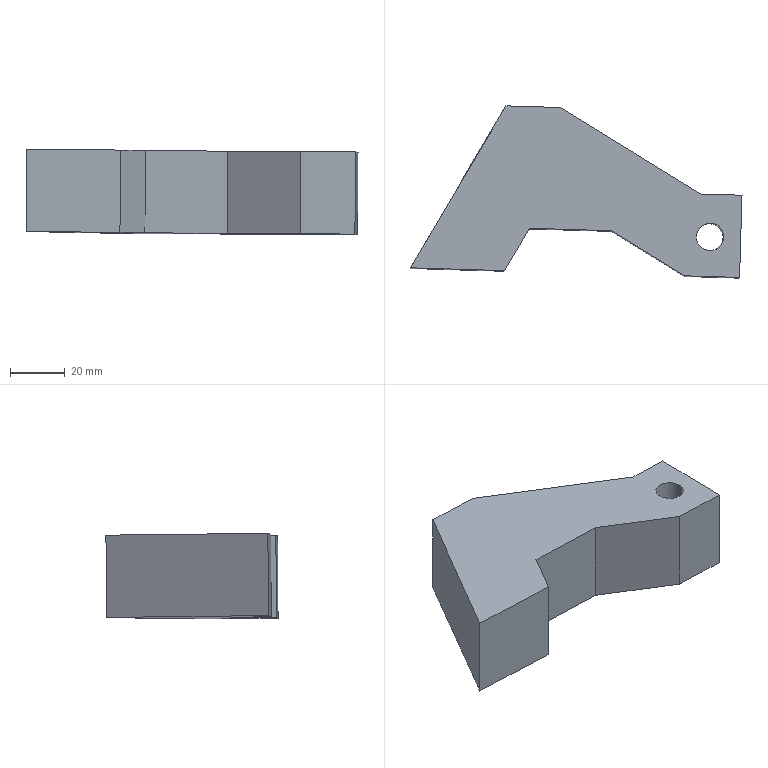Component | NX | M1002_AGO13_P09_757058_P01 | 1 solid | 13 faces | box 121.07 x 62.76 x 31.13 mm | volume 124638 mm3 | plane 12 | cylinder 1 | commonest cylinder face diameters 10 x1
STEP:
#1=CARTESIAN_POINT('',(0.,0.,0.));
#2=DIRECTION('',(0.,0.,1.));
#3=DIRECTION('',(1.,0.,0.));
#4=AXIS2_PLACEMENT_3D('',#1,#2,#3);
#5=CARTESIAN_POINT('',(-375.468,-402.725,117.7));
#6=VERTEX_POINT('',#5);
#7=CARTESIAN_POINT('',(-374.576,-372.739,117.492));
#8=VERTEX_POINT('',#7);
#9=CARTESIAN_POINT('',(-375.468,-402.725,117.7));
#10=DIRECTION('',(0.02973,0.9995,-0.006913));
#11=VECTOR('',#10,1.);
#12=LINE('',#9,#11);
#13=CARTESIAN_POINT('',(-375.23,-402.525,147.698));
#14=DIRECTION('',(-0.9995,0.02978,0.007726));
#15=DIRECTION('',(0.007929,0.00668,0.9999));
#16=AXIS2_PLACEMENT_3D('',#13,#14,#15);
#17=PLANE('',#16);
#18=CARTESIAN_POINT('',(-30.,-0.));
#19=DIRECTION('',(0.,1.));
#20=VECTOR('',#19,1.);
#21=LINE('',#18,#20);
#22=(GEOMETRIC_REPRESENTATION_CONTEXT(2)PARAMETRIC_REPRESENTATION_CONTEXT()REPRESENTATION_CONTEXT('',''));
#23=DEFINITIONAL_REPRESENTATION('',(#21),#22);
#24=PCURVE('',#17,#23);
#25=CARTESIAN_POINT('',(-386.232,-387.898,117.686));
#26=DIRECTION('',(0.007929,0.00668,0.9999));
#27=DIRECTION('',(0.9995,-0.02978,-0.007726));
#28=AXIS2_PLACEMENT_3D('',#25,#26,#27);
#29=PLANE('',#28);
#30=CARTESIAN_POINT('',(11.2,-14.5));
#31=DIRECTION('',(-0.,1.));
#32=VECTOR('',#31,1.);
#33=LINE('',#30,#32);
#34=(GEOMETRIC_REPRESENTATION_CONTEXT(2)PARAMETRIC_REPRESENTATION_CONTEXT()REPRESENTATION_CONTEXT('',''));
#35=DEFINITIONAL_REPRESENTATION('',(#33),#34);
#36=PCURVE('',#29,#35);
#37=SURFACE_CURVE('',#12,(#24,#36),.PCURVE_S1.);
#38=EDGE_CURVE('',#6,#8,#37,.T.);
#39=ORIENTED_EDGE('',*,*,#38,.T.);
#40=CARTESIAN_POINT('',(-374.338,-372.539,147.491));
#41=VERTEX_POINT('',#40);
#42=CARTESIAN_POINT('',(-374.338,-372.539,147.491));
#43=DIRECTION('',(-0.007929,-0.00668,-0.9999));
#44=VECTOR('',#43,1.);
#45=LINE('',#42,#44);
#46=CARTESIAN_POINT('',(-0.,30.));
#47=DIRECTION('',(-1.,0.));
#48=VECTOR('',#47,1.);
#49=LINE('',#46,#48);
#50=(GEOMETRIC_REPRESENTATION_CONTEXT(2)PARAMETRIC_REPRESENTATION_CONTEXT()REPRESENTATION_CONTEXT('',''));
#51=DEFINITIONAL_REPRESENTATION('',(#49),#50);
#52=PCURVE('',#17,#51);
#53=CARTESIAN_POINT('',(-374.338,-372.539,147.491));
#54=DIRECTION('',(-0.02973,-0.9995,0.006913));
#55=DIRECTION('',(0.9995,-0.02978,-0.007726));
#56=AXIS2_PLACEMENT_3D('',#53,#54,#55);
#57=PLANE('',#56);
#58=CARTESIAN_POINT('',(0.,0.));
#59=DIRECTION('',(-0.,-1.));
#60=VECTOR('',#59,1.);
#61=LINE('',#58,#60);
#62=(GEOMETRIC_REPRESENTATION_CONTEXT(2)PARAMETRIC_REPRESENTATION_CONTEXT()REPRESENTATION_CONTEXT('',''));
#63=DEFINITIONAL_REPRESENTATION('',(#61),#62);
#64=PCURVE('',#57,#63);
#65=SURFACE_CURVE('',#45,(#52,#64),.PCURVE_S1.);
#66=EDGE_CURVE('',#41,#8,#65,.T.);
#67=ORIENTED_EDGE('',*,*,#66,.F.);
#68=CARTESIAN_POINT('',(-375.23,-402.525,147.698));
#69=VERTEX_POINT('',#68);
#70=CARTESIAN_POINT('',(-375.23,-402.525,147.698));
#71=DIRECTION('',(0.02973,0.9995,-0.006913));
#72=VECTOR('',#71,1.);
#73=LINE('',#70,#72);
#74=CARTESIAN_POINT('',(0.,0.));
#75=DIRECTION('',(0.,1.));
#76=VECTOR('',#75,1.);
#77=LINE('',#74,#76);
#78=(GEOMETRIC_REPRESENTATION_CONTEXT(2)PARAMETRIC_REPRESENTATION_CONTEXT()REPRESENTATION_CONTEXT('',''));
#79=DEFINITIONAL_REPRESENTATION('',(#77),#78);
#80=PCURVE('',#17,#79);
#81=CARTESIAN_POINT('',(-385.994,-387.698,147.684));
#82=DIRECTION('',(0.007929,0.00668,0.9999));
#83=DIRECTION('',(0.9995,-0.02978,-0.007726));
#84=AXIS2_PLACEMENT_3D('',#81,#82,#83);
#85=PLANE('',#84);
#86=CARTESIAN_POINT('',(11.2,-14.5));
#87=DIRECTION('',(-0.,1.));
#88=VECTOR('',#87,1.);
#89=LINE('',#86,#88);
#90=(GEOMETRIC_REPRESENTATION_CONTEXT(2)PARAMETRIC_REPRESENTATION_CONTEXT()REPRESENTATION_CONTEXT('',''));
#91=DEFINITIONAL_REPRESENTATION('',(#89),#90);
#92=PCURVE('',#85,#91);
#93=SURFACE_CURVE('',#73,(#80,#92),.PCURVE_S1.);
#94=EDGE_CURVE('',#69,#41,#93,.T.);
#95=ORIENTED_EDGE('',*,*,#94,.F.);
#96=CARTESIAN_POINT('',(-375.23,-402.525,147.698));
#97=DIRECTION('',(-0.007929,-0.00668,-0.9999));
#98=VECTOR('',#97,1.);
#99=LINE('',#96,#98);
#100=CARTESIAN_POINT('',(0.,0.));
#101=DIRECTION('',(-1.,0.));
#102=VECTOR('',#101,1.);
#103=LINE('',#100,#102);
#104=(GEOMETRIC_REPRESENTATION_CONTEXT(2)PARAMETRIC_REPRESENTATION_CONTEXT()REPRESENTATION_CONTEXT('',''));
#105=DEFINITIONAL_REPRESENTATION('',(#103),#104);
#106=PCURVE('',#17,#105);
#107=CARTESIAN_POINT('',(-395.221,-401.929,147.853));
#108=DIRECTION('',(0.02973,0.9995,-0.006913));
#109=DIRECTION('',(-0.9995,0.02978,0.007726));
#110=AXIS2_PLACEMENT_3D('',#107,#108,#109);
#111=PLANE('',#110);
#112=CARTESIAN_POINT('',(-20.,-0.));
#113=DIRECTION('',(0.,-1.));
#114=VECTOR('',#113,1.);
#115=LINE('',#112,#114);
#116=(GEOMETRIC_REPRESENTATION_CONTEXT(2)PARAMETRIC_REPRESENTATION_CONTEXT()REPRESENTATION_CONTEXT('',''));
#117=DEFINITIONAL_REPRESENTATION('',(#115),#116);
#118=PCURVE('',#111,#117);
#119=SURFACE_CURVE('',#99,(#106,#118),.PCURVE_S1.);
#120=EDGE_CURVE('',#69,#6,#119,.T.);
#121=ORIENTED_EDGE('',*,*,#120,.T.);
#122=EDGE_LOOP('',(#39,#67,#95,#121));
#123=FACE_BOUND('',#122,.T.);
#124=ADVANCED_FACE('',(#123),#17,.F.);
#125=CARTESIAN_POINT('',(-389.569,-372.292,117.608));
#126=VERTEX_POINT('',#125);
#127=CARTESIAN_POINT('',(-374.576,-372.739,117.492));
#128=DIRECTION('',(-0.9995,0.02978,0.007726));
#129=VECTOR('',#128,1.);
#130=LINE('',#127,#129);
#131=CARTESIAN_POINT('',(-0.,-30.));
#132=DIRECTION('',(-1.,0.));
#133=VECTOR('',#132,1.);
#134=LINE('',#131,#133);
#135=(GEOMETRIC_REPRESENTATION_CONTEXT(2)PARAMETRIC_REPRESENTATION_CONTEXT()REPRESENTATION_CONTEXT('',''));
#136=DEFINITIONAL_REPRESENTATION('',(#134),#135);
#137=PCURVE('',#57,#136);
#138=CARTESIAN_POINT('',(11.2,15.5));
#139=DIRECTION('',(-1.,-0.));
#140=VECTOR('',#139,1.);
#141=LINE('',#138,#140);
#142=(GEOMETRIC_REPRESENTATION_CONTEXT(2)PARAMETRIC_REPRESENTATION_CONTEXT()REPRESENTATION_CONTEXT('',''));
#143=DEFINITIONAL_REPRESENTATION('',(#141),#142);
#144=PCURVE('',#29,#143);
#145=SURFACE_CURVE('',#130,(#137,#144),.PCURVE_S1.);
#146=EDGE_CURVE('',#8,#126,#145,.T.);
#147=ORIENTED_EDGE('',*,*,#146,.T.);
#148=CARTESIAN_POINT('',(-389.331,-372.092,147.607));
#149=VERTEX_POINT('',#148);
#150=CARTESIAN_POINT('',(-389.331,-372.092,147.607));
#151=DIRECTION('',(-0.007929,-0.00668,-0.9999));
#152=VECTOR('',#151,1.);
#153=LINE('',#150,#152);
#154=CARTESIAN_POINT('',(-15.,0.));
#155=DIRECTION('',(-0.,-1.));
#156=VECTOR('',#155,1.);
#157=LINE('',#154,#156);
#158=(GEOMETRIC_REPRESENTATION_CONTEXT(2)PARAMETRIC_REPRESENTATION_CONTEXT()REPRESENTATION_CONTEXT('',''));
#159=DEFINITIONAL_REPRESENTATION('',(#157),#158);
#160=PCURVE('',#57,#159);
#161=CARTESIAN_POINT('',(-389.331,-372.092,147.607));
#162=DIRECTION('',(-0.5252,-0.8509,0.009849));
#163=DIRECTION('',(0.8509,-0.5253,-0.003238));
#164=AXIS2_PLACEMENT_3D('',#161,#162,#163);
#165=PLANE('',#164);
#166=CARTESIAN_POINT('',(0.,0.));
#167=DIRECTION('',(0.,-1.));
#168=VECTOR('',#167,1.);
#169=LINE('',#166,#168);
#170=(GEOMETRIC_REPRESENTATION_CONTEXT(2)PARAMETRIC_REPRESENTATION_CONTEXT()REPRESENTATION_CONTEXT('',''));
#171=DEFINITIONAL_REPRESENTATION('',(#169),#170);
#172=PCURVE('',#165,#171);
#173=SURFACE_CURVE('',#153,(#160,#172),.PCURVE_S1.);
#174=EDGE_CURVE('',#149,#126,#173,.T.);
#175=ORIENTED_EDGE('',*,*,#174,.F.);
#176=CARTESIAN_POINT('',(-374.338,-372.539,147.491));
#177=DIRECTION('',(-0.9995,0.02978,0.007726));
#178=VECTOR('',#177,1.);
#179=LINE('',#176,#178);
#180=CARTESIAN_POINT('',(0.,0.));
#181=DIRECTION('',(-1.,0.));
#182=VECTOR('',#181,1.);
#183=LINE('',#180,#182);
#184=(GEOMETRIC_REPRESENTATION_CONTEXT(2)PARAMETRIC_REPRESENTATION_CONTEXT()REPRESENTATION_CONTEXT('',''));
#185=DEFINITIONAL_REPRESENTATION('',(#183),#184);
#186=PCURVE('',#57,#185);
#187=CARTESIAN_POINT('',(11.2,15.5));
#188=DIRECTION('',(-1.,-0.));
#189=VECTOR('',#188,1.);
#190=LINE('',#187,#189);
#191=(GEOMETRIC_REPRESENTATION_CONTEXT(2)PARAMETRIC_REPRESENTATION_CONTEXT()REPRESENTATION_CONTEXT('',''));
#192=DEFINITIONAL_REPRESENTATION('',(#190),#191);
#193=PCURVE('',#85,#192);
#194=SURFACE_CURVE('',#179,(#186,#193),.PCURVE_S1.);
#195=EDGE_CURVE('',#41,#149,#194,.T.);
#196=ORIENTED_EDGE('',*,*,#195,.F.);
#197=ORIENTED_EDGE('',*,*,#66,.T.);
#198=EDGE_LOOP('',(#147,#175,#196,#197));
#199=FACE_BOUND('',#198,.T.);
#200=ADVANCED_FACE('',(#199),#57,.F.);
#201=CARTESIAN_POINT('',(-440.653,-340.758,117.803));
#202=VERTEX_POINT('',#201);
#203=CARTESIAN_POINT('',(-389.569,-372.292,117.608));
#204=DIRECTION('',(-0.8509,0.5253,0.003238));
#205=VECTOR('',#204,1.);
#206=LINE('',#203,#205);
#207=CARTESIAN_POINT('',(0.,-30.));
#208=DIRECTION('',(-1.,-0.));
#209=VECTOR('',#208,1.);
#210=LINE('',#207,#209);
#211=(GEOMETRIC_REPRESENTATION_CONTEXT(2)PARAMETRIC_REPRESENTATION_CONTEXT()REPRESENTATION_CONTEXT('',''));
#212=DEFINITIONAL_REPRESENTATION('',(#210),#211);
#213=PCURVE('',#165,#212);
#214=CARTESIAN_POINT('',(-3.8,15.5));
#215=DIRECTION('',(-0.8662,0.4997));
#216=VECTOR('',#215,1.);
#217=LINE('',#214,#216);
#218=(GEOMETRIC_REPRESENTATION_CONTEXT(2)PARAMETRIC_REPRESENTATION_CONTEXT()REPRESENTATION_CONTEXT('',''));
#219=DEFINITIONAL_REPRESENTATION('',(#217),#218);
#220=PCURVE('',#29,#219);
#221=SURFACE_CURVE('',#206,(#213,#220),.PCURVE_S1.);
#222=EDGE_CURVE('',#126,#202,#221,.T.);
#223=ORIENTED_EDGE('',*,*,#222,.T.);
#224=CARTESIAN_POINT('',(-440.415,-340.557,147.801));
#225=VERTEX_POINT('',#224);
#226=CARTESIAN_POINT('',(-440.415,-340.557,147.801));
#227=DIRECTION('',(-0.007929,-0.00668,-0.9999));
#228=VECTOR('',#227,1.);
#229=LINE('',#226,#228);
#230=CARTESIAN_POINT('',(-60.033,-0.));
#231=DIRECTION('',(0.,-1.));
#232=VECTOR('',#231,1.);
#233=LINE('',#230,#232);
#234=(GEOMETRIC_REPRESENTATION_CONTEXT(2)PARAMETRIC_REPRESENTATION_CONTEXT()REPRESENTATION_CONTEXT('',''));
#235=DEFINITIONAL_REPRESENTATION('',(#233),#234);
#236=PCURVE('',#165,#235);
#237=CARTESIAN_POINT('',(-440.415,-340.557,147.801));
#238=DIRECTION('',(-0.02973,-0.9995,0.006913));
#239=DIRECTION('',(0.9995,-0.02978,-0.007726));
#240=AXIS2_PLACEMENT_3D('',#237,#238,#239);
#241=PLANE('',#240);
#242=CARTESIAN_POINT('',(0.,0.));
#243=DIRECTION('',(-0.,-1.));
#244=VECTOR('',#243,1.);
#245=LINE('',#242,#244);
#246=(GEOMETRIC_REPRESENTATION_CONTEXT(2)PARAMETRIC_REPRESENTATION_CONTEXT()REPRESENTATION_CONTEXT('',''));
#247=DEFINITIONAL_REPRESENTATION('',(#245),#246);
#248=PCURVE('',#241,#247);
#249=SURFACE_CURVE('',#229,(#236,#248),.PCURVE_S1.);
#250=EDGE_CURVE('',#225,#202,#249,.T.);
#251=ORIENTED_EDGE('',*,*,#250,.F.);
#252=CARTESIAN_POINT('',(-389.331,-372.092,147.607));
#253=DIRECTION('',(-0.8509,0.5253,0.003238));
#254=VECTOR('',#253,1.);
#255=LINE('',#252,#254);
#256=CARTESIAN_POINT('',(0.,0.));
#257=DIRECTION('',(-1.,-0.));
#258=VECTOR('',#257,1.);
#259=LINE('',#256,#258);
#260=(GEOMETRIC_REPRESENTATION_CONTEXT(2)PARAMETRIC_REPRESENTATION_CONTEXT()REPRESENTATION_CONTEXT('',''));
#261=DEFINITIONAL_REPRESENTATION('',(#259),#260);
#262=PCURVE('',#165,#261);
#263=CARTESIAN_POINT('',(-3.8,15.5));
#264=DIRECTION('',(-0.8662,0.4997));
#265=VECTOR('',#264,1.);
#266=LINE('',#263,#265);
#267=(GEOMETRIC_REPRESENTATION_CONTEXT(2)PARAMETRIC_REPRESENTATION_CONTEXT()REPRESENTATION_CONTEXT('',''));
#268=DEFINITIONAL_REPRESENTATION('',(#266),#267);
#269=PCURVE('',#85,#268);
#270=SURFACE_CURVE('',#255,(#262,#269),.PCURVE_S1.);
#271=EDGE_CURVE('',#149,#225,#270,.T.);
#272=ORIENTED_EDGE('',*,*,#271,.F.);
#273=ORIENTED_EDGE('',*,*,#174,.T.);
#274=EDGE_LOOP('',(#223,#251,#272,#273));
#275=FACE_BOUND('',#274,.T.);
#276=ADVANCED_FACE('',(#275),#165,.F.);
#277=CARTESIAN_POINT('',(-460.643,-340.162,117.957));
#278=VERTEX_POINT('',#277);
#279=CARTESIAN_POINT('',(-440.653,-340.758,117.803));
#280=DIRECTION('',(-0.9995,0.02978,0.007726));
#281=VECTOR('',#280,1.);
#282=LINE('',#279,#281);
#283=CARTESIAN_POINT('',(-0.,-30.));
#284=DIRECTION('',(-1.,0.));
#285=VECTOR('',#284,1.);
#286=LINE('',#283,#285);
#287=(GEOMETRIC_REPRESENTATION_CONTEXT(2)PARAMETRIC_REPRESENTATION_CONTEXT()REPRESENTATION_CONTEXT('',''));
#288=DEFINITIONAL_REPRESENTATION('',(#286),#287);
#289=PCURVE('',#241,#288);
#290=CARTESIAN_POINT('',(-55.8,45.5));
#291=DIRECTION('',(-1.,-0.));
#292=VECTOR('',#291,1.);
#293=LINE('',#290,#292);
#294=(GEOMETRIC_REPRESENTATION_CONTEXT(2)PARAMETRIC_REPRESENTATION_CONTEXT()REPRESENTATION_CONTEXT('',''));
#295=DEFINITIONAL_REPRESENTATION('',(#293),#294);
#296=PCURVE('',#29,#295);
#297=SURFACE_CURVE('',#282,(#289,#296),.PCURVE_S1.);
#298=EDGE_CURVE('',#202,#278,#297,.T.);
#299=ORIENTED_EDGE('',*,*,#298,.T.);
#300=CARTESIAN_POINT('',(-460.405,-339.962,147.956));
#301=VERTEX_POINT('',#300);
#302=CARTESIAN_POINT('',(-460.405,-339.962,147.956));
#303=DIRECTION('',(-0.007929,-0.00668,-0.9999));
#304=VECTOR('',#303,1.);
#305=LINE('',#302,#304);
#306=CARTESIAN_POINT('',(-20.,-0.));
#307=DIRECTION('',(-0.,-1.));
#308=VECTOR('',#307,1.);
#309=LINE('',#306,#308);
#310=(GEOMETRIC_REPRESENTATION_CONTEXT(2)PARAMETRIC_REPRESENTATION_CONTEXT()REPRESENTATION_CONTEXT('',''));
#311=DEFINITIONAL_REPRESENTATION('',(#309),#310);
#312=PCURVE('',#241,#311);
#313=CARTESIAN_POINT('',(-460.405,-339.962,147.956));
#314=DIRECTION('',(0.8617,-0.5074,-0.003443));
#315=DIRECTION('',(0.5073,0.8617,-0.00978));
#316=AXIS2_PLACEMENT_3D('',#313,#314,#315);
#317=PLANE('',#316);
#318=CARTESIAN_POINT('',(0.,0.));
#319=DIRECTION('',(0.,-1.));
#320=VECTOR('',#319,1.);
#321=LINE('',#318,#320);
#322=(GEOMETRIC_REPRESENTATION_CONTEXT(2)PARAMETRIC_REPRESENTATION_CONTEXT()REPRESENTATION_CONTEXT('',''));
#323=DEFINITIONAL_REPRESENTATION('',(#321),#322);
#324=PCURVE('',#317,#323);
#325=SURFACE_CURVE('',#305,(#312,#324),.PCURVE_S1.);
#326=EDGE_CURVE('',#301,#278,#325,.T.);
#327=ORIENTED_EDGE('',*,*,#326,.F.);
#328=CARTESIAN_POINT('',(-440.415,-340.557,147.801));
#329=DIRECTION('',(-0.9995,0.02978,0.007726));
#330=VECTOR('',#329,1.);
#331=LINE('',#328,#330);
#332=CARTESIAN_POINT('',(0.,0.));
#333=DIRECTION('',(-1.,0.));
#334=VECTOR('',#333,1.);
#335=LINE('',#332,#334);
#336=(GEOMETRIC_REPRESENTATION_CONTEXT(2)PARAMETRIC_REPRESENTATION_CONTEXT()REPRESENTATION_CONTEXT('',''));
#337=DEFINITIONAL_REPRESENTATION('',(#335),#336);
#338=PCURVE('',#241,#337);
#339=CARTESIAN_POINT('',(-55.8,45.5));
#340=DIRECTION('',(-1.,-0.));
#341=VECTOR('',#340,1.);
#342=LINE('',#339,#341);
#343=(GEOMETRIC_REPRESENTATION_CONTEXT(2)PARAMETRIC_REPRESENTATION_CONTEXT()REPRESENTATION_CONTEXT('',''));
#344=DEFINITIONAL_REPRESENTATION('',(#342),#343);
#345=PCURVE('',#85,#344);
#346=SURFACE_CURVE('',#331,(#338,#345),.PCURVE_S1.);
#347=EDGE_CURVE('',#225,#301,#346,.T.);
#348=ORIENTED_EDGE('',*,*,#347,.F.);
#349=ORIENTED_EDGE('',*,*,#250,.T.);
#350=EDGE_LOOP('',(#299,#327,#348,#349));
#351=FACE_BOUND('',#350,.T.);
#352=ADVANCED_FACE('',(#351),#241,.F.);
#353=CARTESIAN_POINT('',(-495.413,-399.217,118.627));
#354=VERTEX_POINT('',#353);
#355=CARTESIAN_POINT('',(-460.643,-340.162,117.957));
#356=DIRECTION('',(-0.5073,-0.8617,0.00978));
#357=VECTOR('',#356,1.);
#358=LINE('',#355,#357);
#359=CARTESIAN_POINT('',(0.,-30.));
#360=DIRECTION('',(-1.,-0.));
#361=VECTOR('',#360,1.);
#362=LINE('',#359,#361);
#363=(GEOMETRIC_REPRESENTATION_CONTEXT(2)PARAMETRIC_REPRESENTATION_CONTEXT()REPRESENTATION_CONTEXT('',''));
#364=DEFINITIONAL_REPRESENTATION('',(#362),#363);
#365=PCURVE('',#317,#364);
#366=CARTESIAN_POINT('',(-75.8,45.5));
#367=DIRECTION('',(-0.4815,-0.8764));
#368=VECTOR('',#367,1.);
#369=LINE('',#366,#368);
#370=(GEOMETRIC_REPRESENTATION_CONTEXT(2)PARAMETRIC_REPRESENTATION_CONTEXT()REPRESENTATION_CONTEXT('',''));
#371=DEFINITIONAL_REPRESENTATION('',(#369),#370);
#372=PCURVE('',#29,#371);
#373=SURFACE_CURVE('',#358,(#365,#372),.PCURVE_S1.);
#374=EDGE_CURVE('',#278,#354,#373,.T.);
#375=ORIENTED_EDGE('',*,*,#374,.T.);
#376=CARTESIAN_POINT('',(-495.175,-399.017,148.626));
#377=VERTEX_POINT('',#376);
#378=CARTESIAN_POINT('',(-495.175,-399.017,148.626));
#379=DIRECTION('',(-0.007929,-0.00668,-0.9999));
#380=VECTOR('',#379,1.);
#381=LINE('',#378,#380);
#382=CARTESIAN_POINT('',(-68.534,-0.));
#383=DIRECTION('',(0.,-1.));
#384=VECTOR('',#383,1.);
#385=LINE('',#382,#384);
#386=(GEOMETRIC_REPRESENTATION_CONTEXT(2)PARAMETRIC_REPRESENTATION_CONTEXT()REPRESENTATION_CONTEXT('',''));
#387=DEFINITIONAL_REPRESENTATION('',(#385),#386);
#388=PCURVE('',#317,#387);
#389=CARTESIAN_POINT('',(-495.175,-399.017,148.626));
#390=DIRECTION('',(0.02973,0.9995,-0.006913));
#391=DIRECTION('',(-0.9995,0.02978,0.007726));
#392=AXIS2_PLACEMENT_3D('',#389,#390,#391);
#393=PLANE('',#392);
#394=CARTESIAN_POINT('',(0.,0.));
#395=DIRECTION('',(0.,-1.));
#396=VECTOR('',#395,1.);
#397=LINE('',#394,#396);
#398=(GEOMETRIC_REPRESENTATION_CONTEXT(2)PARAMETRIC_REPRESENTATION_CONTEXT()REPRESENTATION_CONTEXT('',''));
#399=DEFINITIONAL_REPRESENTATION('',(#397),#398);
#400=PCURVE('',#393,#399);
#401=SURFACE_CURVE('',#381,(#388,#400),.PCURVE_S1.);
#402=EDGE_CURVE('',#377,#354,#401,.T.);
#403=ORIENTED_EDGE('',*,*,#402,.F.);
#404=CARTESIAN_POINT('',(-460.405,-339.962,147.956));
#405=DIRECTION('',(-0.5073,-0.8617,0.00978));
#406=VECTOR('',#405,1.);
#407=LINE('',#404,#406);
#408=CARTESIAN_POINT('',(0.,0.));
#409=DIRECTION('',(-1.,-0.));
#410=VECTOR('',#409,1.);
#411=LINE('',#408,#410);
#412=(GEOMETRIC_REPRESENTATION_CONTEXT(2)PARAMETRIC_REPRESENTATION_CONTEXT()REPRESENTATION_CONTEXT('',''));
#413=DEFINITIONAL_REPRESENTATION('',(#411),#412);
#414=PCURVE('',#317,#413);
#415=CARTESIAN_POINT('',(-75.8,45.5));
#416=DIRECTION('',(-0.4815,-0.8764));
#417=VECTOR('',#416,1.);
#418=LINE('',#415,#417);
#419=(GEOMETRIC_REPRESENTATION_CONTEXT(2)PARAMETRIC_REPRESENTATION_CONTEXT()REPRESENTATION_CONTEXT('',''));
#420=DEFINITIONAL_REPRESENTATION('',(#418),#419);
#421=PCURVE('',#85,#420);
#422=SURFACE_CURVE('',#407,(#414,#421),.PCURVE_S1.);
#423=EDGE_CURVE('',#301,#377,#422,.T.);
#424=ORIENTED_EDGE('',*,*,#423,.F.);
#425=ORIENTED_EDGE('',*,*,#326,.T.);
#426=EDGE_LOOP('',(#375,#403,#424,#425));
#427=FACE_BOUND('',#426,.T.);
#428=ADVANCED_FACE('',(#427),#317,.F.);
#429=CARTESIAN_POINT('',(-461.155,-400.238,118.363));
#430=VERTEX_POINT('',#429);
#431=CARTESIAN_POINT('',(-495.413,-399.217,118.627));
#432=DIRECTION('',(0.9995,-0.02978,-0.007726));
#433=VECTOR('',#432,1.);
#434=LINE('',#431,#433);
#435=CARTESIAN_POINT('',(0.,-30.));
#436=DIRECTION('',(-1.,-0.));
#437=VECTOR('',#436,1.);
#438=LINE('',#435,#437);
#439=(GEOMETRIC_REPRESENTATION_CONTEXT(2)PARAMETRIC_REPRESENTATION_CONTEXT()REPRESENTATION_CONTEXT('',''));
#440=DEFINITIONAL_REPRESENTATION('',(#438),#439);
#441=PCURVE('',#393,#440);
#442=CARTESIAN_POINT('',(-108.8,-14.565));
#443=DIRECTION('',(1.,0.));
#444=VECTOR('',#443,1.);
#445=LINE('',#442,#444);
#446=(GEOMETRIC_REPRESENTATION_CONTEXT(2)PARAMETRIC_REPRESENTATION_CONTEXT()REPRESENTATION_CONTEXT('',''));
#447=DEFINITIONAL_REPRESENTATION('',(#445),#446);
#448=PCURVE('',#29,#447);
#449=SURFACE_CURVE('',#434,(#441,#448),.PCURVE_S1.);
#450=EDGE_CURVE('',#354,#430,#449,.T.);
#451=ORIENTED_EDGE('',*,*,#450,.T.);
#452=CARTESIAN_POINT('',(-460.917,-400.037,148.361));
#453=VERTEX_POINT('',#452);
#454=CARTESIAN_POINT('',(-460.917,-400.037,148.361));
#455=DIRECTION('',(-0.007929,-0.00668,-0.9999));
#456=VECTOR('',#455,1.);
#457=LINE('',#454,#456);
#458=CARTESIAN_POINT('',(-34.274,0.));
#459=DIRECTION('',(0.,-1.));
#460=VECTOR('',#459,1.);
#461=LINE('',#458,#460);
#462=(GEOMETRIC_REPRESENTATION_CONTEXT(2)PARAMETRIC_REPRESENTATION_CONTEXT()REPRESENTATION_CONTEXT('',''));
#463=DEFINITIONAL_REPRESENTATION('',(#461),#462);
#464=PCURVE('',#393,#463);
#465=CARTESIAN_POINT('',(-460.917,-400.037,148.361));
#466=DIRECTION('',(-0.8617,0.5074,0.003443));
#467=DIRECTION('',(-0.5073,-0.8617,0.00978));
#468=AXIS2_PLACEMENT_3D('',#465,#466,#467);
#469=PLANE('',#468);
#470=CARTESIAN_POINT('',(0.,0.));
#471=DIRECTION('',(-0.,-1.));
#472=VECTOR('',#471,1.);
#473=LINE('',#470,#472);
#474=(GEOMETRIC_REPRESENTATION_CONTEXT(2)PARAMETRIC_REPRESENTATION_CONTEXT()REPRESENTATION_CONTEXT('',''));
#475=DEFINITIONAL_REPRESENTATION('',(#473),#474);
#476=PCURVE('',#469,#475);
#477=SURFACE_CURVE('',#457,(#464,#476),.PCURVE_S1.);
#478=EDGE_CURVE('',#453,#430,#477,.T.);
#479=ORIENTED_EDGE('',*,*,#478,.F.);
#480=CARTESIAN_POINT('',(-495.175,-399.017,148.626));
#481=DIRECTION('',(0.9995,-0.02978,-0.007726));
#482=VECTOR('',#481,1.);
#483=LINE('',#480,#482);
#484=CARTESIAN_POINT('',(0.,0.));
#485=DIRECTION('',(-1.,-0.));
#486=VECTOR('',#485,1.);
#487=LINE('',#484,#486);
#488=(GEOMETRIC_REPRESENTATION_CONTEXT(2)PARAMETRIC_REPRESENTATION_CONTEXT()REPRESENTATION_CONTEXT('',''));
#489=DEFINITIONAL_REPRESENTATION('',(#487),#488);
#490=PCURVE('',#393,#489);
#491=CARTESIAN_POINT('',(-108.8,-14.565));
#492=DIRECTION('',(1.,0.));
#493=VECTOR('',#492,1.);
#494=LINE('',#491,#493);
#495=(GEOMETRIC_REPRESENTATION_CONTEXT(2)PARAMETRIC_REPRESENTATION_CONTEXT()REPRESENTATION_CONTEXT('',''));
#496=DEFINITIONAL_REPRESENTATION('',(#494),#495);
#497=PCURVE('',#85,#496);
#498=SURFACE_CURVE('',#483,(#490,#497),.PCURVE_S1.);
#499=EDGE_CURVE('',#377,#453,#498,.T.);
#500=ORIENTED_EDGE('',*,*,#499,.F.);
#501=ORIENTED_EDGE('',*,*,#402,.T.);
#502=EDGE_LOOP('',(#451,#479,#500,#501));
#503=FACE_BOUND('',#502,.T.);
#504=ADVANCED_FACE('',(#503),#393,.F.);
#505=CARTESIAN_POINT('',(-452.067,-384.802,118.187));
#506=VERTEX_POINT('',#505);
#507=CARTESIAN_POINT('',(-461.155,-400.238,118.363));
#508=DIRECTION('',(0.5073,0.8617,-0.00978));
#509=VECTOR('',#508,1.);
#510=LINE('',#507,#509);
#511=CARTESIAN_POINT('',(0.,-30.));
#512=DIRECTION('',(-1.,0.));
#513=VECTOR('',#512,1.);
#514=LINE('',#511,#513);
#515=(GEOMETRIC_REPRESENTATION_CONTEXT(2)PARAMETRIC_REPRESENTATION_CONTEXT()REPRESENTATION_CONTEXT('',''));
#516=DEFINITIONAL_REPRESENTATION('',(#514),#515);
#517=PCURVE('',#469,#516);
#518=CARTESIAN_POINT('',(-74.526,-14.565));
#519=DIRECTION('',(0.4815,0.8764));
#520=VECTOR('',#519,1.);
#521=LINE('',#518,#520);
#522=(GEOMETRIC_REPRESENTATION_CONTEXT(2)PARAMETRIC_REPRESENTATION_CONTEXT()REPRESENTATION_CONTEXT('',''));
#523=DEFINITIONAL_REPRESENTATION('',(#521),#522);
#524=PCURVE('',#29,#523);
#525=SURFACE_CURVE('',#510,(#517,#524),.PCURVE_S1.);
#526=EDGE_CURVE('',#430,#506,#525,.T.);
#527=ORIENTED_EDGE('',*,*,#526,.T.);
#528=CARTESIAN_POINT('',(-451.829,-384.601,148.186));
#529=VERTEX_POINT('',#528);
#530=CARTESIAN_POINT('',(-451.829,-384.601,148.186));
#531=DIRECTION('',(-0.007929,-0.00668,-0.9999));
#532=VECTOR('',#531,1.);
#533=LINE('',#530,#532);
#534=CARTESIAN_POINT('',(-17.913,-0.));
#535=DIRECTION('',(-0.,-1.));
#536=VECTOR('',#535,1.);
#537=LINE('',#534,#536);
#538=(GEOMETRIC_REPRESENTATION_CONTEXT(2)PARAMETRIC_REPRESENTATION_CONTEXT()REPRESENTATION_CONTEXT('',''));
#539=DEFINITIONAL_REPRESENTATION('',(#537),#538);
#540=PCURVE('',#469,#539);
#541=CARTESIAN_POINT('',(-451.829,-384.601,148.186));
#542=DIRECTION('',(0.02973,0.9995,-0.006913));
#543=DIRECTION('',(-0.9995,0.02978,0.007726));
#544=AXIS2_PLACEMENT_3D('',#541,#542,#543);
#545=PLANE('',#544);
#546=CARTESIAN_POINT('',(0.,0.));
#547=DIRECTION('',(0.,-1.));
#548=VECTOR('',#547,1.);
#549=LINE('',#546,#548);
#550=(GEOMETRIC_REPRESENTATION_CONTEXT(2)PARAMETRIC_REPRESENTATION_CONTEXT()REPRESENTATION_CONTEXT('',''));
#551=DEFINITIONAL_REPRESENTATION('',(#549),#550);
#552=PCURVE('',#545,#551);
#553=SURFACE_CURVE('',#533,(#540,#552),.PCURVE_S1.);
#554=EDGE_CURVE('',#529,#506,#553,.T.);
#555=ORIENTED_EDGE('',*,*,#554,.F.);
#556=CARTESIAN_POINT('',(-460.917,-400.037,148.361));
#557=DIRECTION('',(0.5073,0.8617,-0.00978));
#558=VECTOR('',#557,1.);
#559=LINE('',#556,#558);
#560=CARTESIAN_POINT('',(0.,0.));
#561=DIRECTION('',(-1.,0.));
#562=VECTOR('',#561,1.);
#563=LINE('',#560,#562);
#564=(GEOMETRIC_REPRESENTATION_CONTEXT(2)PARAMETRIC_REPRESENTATION_CONTEXT()REPRESENTATION_CONTEXT('',''));
#565=DEFINITIONAL_REPRESENTATION('',(#563),#564);
#566=PCURVE('',#469,#565);
#567=CARTESIAN_POINT('',(-74.526,-14.565));
#568=DIRECTION('',(0.4815,0.8764));
#569=VECTOR('',#568,1.);
#570=LINE('',#567,#569);
#571=(GEOMETRIC_REPRESENTATION_CONTEXT(2)PARAMETRIC_REPRESENTATION_CONTEXT()REPRESENTATION_CONTEXT('',''));
#572=DEFINITIONAL_REPRESENTATION('',(#570),#571);
#573=PCURVE('',#85,#572);
#574=SURFACE_CURVE('',#559,(#566,#573),.PCURVE_S1.);
#575=EDGE_CURVE('',#453,#529,#574,.T.);
#576=ORIENTED_EDGE('',*,*,#575,.F.);
#577=ORIENTED_EDGE('',*,*,#478,.T.);
#578=EDGE_LOOP('',(#527,#555,#576,#577));
#579=FACE_BOUND('',#578,.T.);
#580=ADVANCED_FACE('',(#579),#469,.F.);
#581=CARTESIAN_POINT('',(-422.081,-385.695,117.956));
#582=VERTEX_POINT('',#581);
#583=CARTESIAN_POINT('',(-452.067,-384.802,118.187));
#584=DIRECTION('',(0.9995,-0.02978,-0.007726));
#585=VECTOR('',#584,1.);
#586=LINE('',#583,#585);
#587=CARTESIAN_POINT('',(0.,-30.));
#588=DIRECTION('',(-1.,-0.));
#589=VECTOR('',#588,1.);
#590=LINE('',#587,#589);
#591=(GEOMETRIC_REPRESENTATION_CONTEXT(2)PARAMETRIC_REPRESENTATION_CONTEXT()REPRESENTATION_CONTEXT('',''));
#592=DEFINITIONAL_REPRESENTATION('',(#590),#591);
#593=PCURVE('',#545,#592);
#594=CARTESIAN_POINT('',(-65.9,1.135));
#595=DIRECTION('',(1.,0.));
#596=VECTOR('',#595,1.);
#597=LINE('',#594,#596);
#598=(GEOMETRIC_REPRESENTATION_CONTEXT(2)PARAMETRIC_REPRESENTATION_CONTEXT()REPRESENTATION_CONTEXT('',''));
#599=DEFINITIONAL_REPRESENTATION('',(#597),#598);
#600=PCURVE('',#29,#599);
#601=SURFACE_CURVE('',#586,(#593,#600),.PCURVE_S1.);
#602=EDGE_CURVE('',#506,#582,#601,.T.);
#603=ORIENTED_EDGE('',*,*,#602,.T.);
#604=CARTESIAN_POINT('',(-421.843,-385.495,147.954));
#605=VERTEX_POINT('',#604);
#606=CARTESIAN_POINT('',(-421.843,-385.495,147.954));
#607=DIRECTION('',(-0.007929,-0.00668,-0.9999));
#608=VECTOR('',#607,1.);
#609=LINE('',#606,#608);
#610=CARTESIAN_POINT('',(-30.,0.));
#611=DIRECTION('',(0.,-1.));
#612=VECTOR('',#611,1.);
#613=LINE('',#610,#612);
#614=(GEOMETRIC_REPRESENTATION_CONTEXT(2)PARAMETRIC_REPRESENTATION_CONTEXT()REPRESENTATION_CONTEXT('',''));
#615=DEFINITIONAL_REPRESENTATION('',(#613),#614);
#616=PCURVE('',#545,#615);
#617=CARTESIAN_POINT('',(-421.843,-385.495,147.954));
#618=DIRECTION('',(0.5252,0.8509,-0.009849));
#619=DIRECTION('',(-0.8509,0.5253,0.003238));
#620=AXIS2_PLACEMENT_3D('',#617,#618,#619);
#621=PLANE('',#620);
#622=CARTESIAN_POINT('',(0.,0.));
#623=DIRECTION('',(0.,-1.));
#624=VECTOR('',#623,1.);
#625=LINE('',#622,#624);
#626=(GEOMETRIC_REPRESENTATION_CONTEXT(2)PARAMETRIC_REPRESENTATION_CONTEXT()REPRESENTATION_CONTEXT('',''));
#627=DEFINITIONAL_REPRESENTATION('',(#625),#626);
#628=PCURVE('',#621,#627);
#629=SURFACE_CURVE('',#609,(#616,#628),.PCURVE_S1.);
#630=EDGE_CURVE('',#605,#582,#629,.T.);
#631=ORIENTED_EDGE('',*,*,#630,.F.);
#632=CARTESIAN_POINT('',(-451.829,-384.601,148.186));
#633=DIRECTION('',(0.9995,-0.02978,-0.007726));
#634=VECTOR('',#633,1.);
#635=LINE('',#632,#634);
#636=CARTESIAN_POINT('',(0.,0.));
#637=DIRECTION('',(-1.,-0.));
#638=VECTOR('',#637,1.);
#639=LINE('',#636,#638);
#640=(GEOMETRIC_REPRESENTATION_CONTEXT(2)PARAMETRIC_REPRESENTATION_CONTEXT()REPRESENTATION_CONTEXT('',''));
#641=DEFINITIONAL_REPRESENTATION('',(#639),#640);
#642=PCURVE('',#545,#641);
#643=CARTESIAN_POINT('',(-65.9,1.135));
#644=DIRECTION('',(1.,0.));
#645=VECTOR('',#644,1.);
#646=LINE('',#643,#645);
#647=(GEOMETRIC_REPRESENTATION_CONTEXT(2)PARAMETRIC_REPRESENTATION_CONTEXT()REPRESENTATION_CONTEXT('',''));
#648=DEFINITIONAL_REPRESENTATION('',(#646),#647);
#649=PCURVE('',#85,#648);
#650=SURFACE_CURVE('',#635,(#642,#649),.PCURVE_S1.);
#651=EDGE_CURVE('',#529,#605,#650,.T.);
#652=ORIENTED_EDGE('',*,*,#651,.F.);
#653=ORIENTED_EDGE('',*,*,#554,.T.);
#654=EDGE_LOOP('',(#603,#631,#652,#653));
#655=FACE_BOUND('',#654,.T.);
#656=ADVANCED_FACE('',(#655),#545,.F.);
#657=CARTESIAN_POINT('',(-395.459,-402.13,117.854));
#658=VERTEX_POINT('',#657);
#659=CARTESIAN_POINT('',(-422.081,-385.695,117.956));
#660=DIRECTION('',(0.8509,-0.5253,-0.003238));
#661=VECTOR('',#660,1.);
#662=LINE('',#659,#661);
#663=CARTESIAN_POINT('',(-0.,-30.));
#664=DIRECTION('',(-1.,0.));
#665=VECTOR('',#664,1.);
#666=LINE('',#663,#665);
#667=(GEOMETRIC_REPRESENTATION_CONTEXT(2)PARAMETRIC_REPRESENTATION_CONTEXT()REPRESENTATION_CONTEXT('',''));
#668=DEFINITIONAL_REPRESENTATION('',(#666),#667);
#669=PCURVE('',#621,#668);
#670=CARTESIAN_POINT('',(-35.9,1.135));
#671=DIRECTION('',(0.8662,-0.4997));
#672=VECTOR('',#671,1.);
#673=LINE('',#670,#672);
#674=(GEOMETRIC_REPRESENTATION_CONTEXT(2)PARAMETRIC_REPRESENTATION_CONTEXT()REPRESENTATION_CONTEXT('',''));
#675=DEFINITIONAL_REPRESENTATION('',(#673),#674);
#676=PCURVE('',#29,#675);
#677=SURFACE_CURVE('',#662,(#669,#676),.PCURVE_S1.);
#678=EDGE_CURVE('',#582,#658,#677,.T.);
#679=ORIENTED_EDGE('',*,*,#678,.T.);
#680=CARTESIAN_POINT('',(-395.221,-401.929,147.853));
#681=VERTEX_POINT('',#680);
#682=CARTESIAN_POINT('',(-395.221,-401.929,147.853));
#683=DIRECTION('',(-0.007929,-0.00668,-0.9999));
#684=VECTOR('',#683,1.);
#685=LINE('',#682,#684);
#686=CARTESIAN_POINT('',(-31.287,0.));
#687=DIRECTION('',(0.,-1.));
#688=VECTOR('',#687,1.);
#689=LINE('',#686,#688);
#690=(GEOMETRIC_REPRESENTATION_CONTEXT(2)PARAMETRIC_REPRESENTATION_CONTEXT()REPRESENTATION_CONTEXT('',''));
#691=DEFINITIONAL_REPRESENTATION('',(#689),#690);
#692=PCURVE('',#621,#691);
#693=CARTESIAN_POINT('',(0.,0.));
#694=DIRECTION('',(0.,-1.));
#695=VECTOR('',#694,1.);
#696=LINE('',#693,#695);
#697=(GEOMETRIC_REPRESENTATION_CONTEXT(2)PARAMETRIC_REPRESENTATION_CONTEXT()REPRESENTATION_CONTEXT('',''));
#698=DEFINITIONAL_REPRESENTATION('',(#696),#697);
#699=PCURVE('',#111,#698);
#700=SURFACE_CURVE('',#685,(#692,#699),.PCURVE_S1.);
#701=EDGE_CURVE('',#681,#658,#700,.T.);
#702=ORIENTED_EDGE('',*,*,#701,.F.);
#703=CARTESIAN_POINT('',(-421.843,-385.495,147.954));
#704=DIRECTION('',(0.8509,-0.5253,-0.003238));
#705=VECTOR('',#704,1.);
#706=LINE('',#703,#705);
#707=CARTESIAN_POINT('',(0.,0.));
#708=DIRECTION('',(-1.,0.));
#709=VECTOR('',#708,1.);
#710=LINE('',#707,#709);
#711=(GEOMETRIC_REPRESENTATION_CONTEXT(2)PARAMETRIC_REPRESENTATION_CONTEXT()REPRESENTATION_CONTEXT('',''));
#712=DEFINITIONAL_REPRESENTATION('',(#710),#711);
#713=PCURVE('',#621,#712);
#714=CARTESIAN_POINT('',(-35.9,1.135));
#715=DIRECTION('',(0.8662,-0.4997));
#716=VECTOR('',#715,1.);
#717=LINE('',#714,#716);
#718=(GEOMETRIC_REPRESENTATION_CONTEXT(2)PARAMETRIC_REPRESENTATION_CONTEXT()REPRESENTATION_CONTEXT('',''));
#719=DEFINITIONAL_REPRESENTATION('',(#717),#718);
#720=PCURVE('',#85,#719);
#721=SURFACE_CURVE('',#706,(#713,#720),.PCURVE_S1.);
#722=EDGE_CURVE('',#605,#681,#721,.T.);
#723=ORIENTED_EDGE('',*,*,#722,.F.);
#724=ORIENTED_EDGE('',*,*,#630,.T.);
#725=EDGE_LOOP('',(#679,#702,#723,#724));
#726=FACE_BOUND('',#725,.T.);
#727=ADVANCED_FACE('',(#726),#621,.F.);
#728=CARTESIAN_POINT('',(-395.459,-402.13,117.854));
#729=DIRECTION('',(0.9995,-0.02978,-0.007726));
#730=VECTOR('',#729,1.);
#731=LINE('',#728,#730);
#732=CARTESIAN_POINT('',(0.,-30.));
#733=DIRECTION('',(-1.,-0.));
#734=VECTOR('',#733,1.);
#735=LINE('',#732,#734);
#736=(GEOMETRIC_REPRESENTATION_CONTEXT(2)PARAMETRIC_REPRESENTATION_CONTEXT()REPRESENTATION_CONTEXT('',''));
#737=DEFINITIONAL_REPRESENTATION('',(#735),#736);
#738=PCURVE('',#111,#737);
#739=CARTESIAN_POINT('',(-8.8,-14.5));
#740=DIRECTION('',(1.,0.));
#741=VECTOR('',#740,1.);
#742=LINE('',#739,#741);
#743=(GEOMETRIC_REPRESENTATION_CONTEXT(2)PARAMETRIC_REPRESENTATION_CONTEXT()REPRESENTATION_CONTEXT('',''));
#744=DEFINITIONAL_REPRESENTATION('',(#742),#743);
#745=PCURVE('',#29,#744);
#746=SURFACE_CURVE('',#731,(#738,#745),.PCURVE_S1.);
#747=EDGE_CURVE('',#658,#6,#746,.T.);
#748=ORIENTED_EDGE('',*,*,#747,.T.);
#749=ORIENTED_EDGE('',*,*,#120,.F.);
#750=CARTESIAN_POINT('',(-395.221,-401.929,147.853));
#751=DIRECTION('',(0.9995,-0.02978,-0.007726));
#752=VECTOR('',#751,1.);
#753=LINE('',#750,#752);
#754=CARTESIAN_POINT('',(0.,0.));
#755=DIRECTION('',(-1.,-0.));
#756=VECTOR('',#755,1.);
#757=LINE('',#754,#756);
#758=(GEOMETRIC_REPRESENTATION_CONTEXT(2)PARAMETRIC_REPRESENTATION_CONTEXT()REPRESENTATION_CONTEXT('',''));
#759=DEFINITIONAL_REPRESENTATION('',(#757),#758);
#760=PCURVE('',#111,#759);
#761=CARTESIAN_POINT('',(-8.8,-14.5));
#762=DIRECTION('',(1.,0.));
#763=VECTOR('',#762,1.);
#764=LINE('',#761,#763);
#765=(GEOMETRIC_REPRESENTATION_CONTEXT(2)PARAMETRIC_REPRESENTATION_CONTEXT()REPRESENTATION_CONTEXT('',''));
#766=DEFINITIONAL_REPRESENTATION('',(#764),#765);
#767=PCURVE('',#85,#766);
#768=SURFACE_CURVE('',#753,(#760,#767),.PCURVE_S1.);
#769=EDGE_CURVE('',#681,#69,#768,.T.);
#770=ORIENTED_EDGE('',*,*,#769,.F.);
#771=ORIENTED_EDGE('',*,*,#701,.T.);
#772=EDGE_LOOP('',(#748,#749,#770,#771));
#773=FACE_BOUND('',#772,.T.);
#774=ADVANCED_FACE('',(#773),#111,.F.);
#775=CARTESIAN_POINT('',(-385.845,-382.7,147.65));
#776=VERTEX_POINT('',#775);
#777=CARTESIAN_POINT('',(-385.994,-387.698,147.684));
#778=DIRECTION('',(0.007929,0.00668,0.9999));
#779=DIRECTION('',(0.02973,0.9995,-0.006913));
#780=AXIS2_PLACEMENT_3D('',#777,#778,#779);
#781=CIRCLE('',#780,5.);
#782=CARTESIAN_POINT('',(-385.994,-387.698,147.684));
#783=DIRECTION('',(-0.007929,-0.00668,-0.9999));
#784=DIRECTION('',(-0.9995,0.02978,0.007726));
#785=AXIS2_PLACEMENT_3D('',#782,#783,#784);
#786=CYLINDRICAL_SURFACE('',#785,5.);
#787=CARTESIAN_POINT('',(7.854,0.));
#788=DIRECTION('',(-1.,0.));
#789=VECTOR('',#788,1.);
#790=LINE('',#787,#789);
#791=(GEOMETRIC_REPRESENTATION_CONTEXT(2)PARAMETRIC_REPRESENTATION_CONTEXT()REPRESENTATION_CONTEXT('',''));
#792=DEFINITIONAL_REPRESENTATION('',(#790),#791);
#793=PCURVE('',#786,#792);
#794=CARTESIAN_POINT('',(0.,0.));
#795=DIRECTION('',(-0.,1.));
#796=AXIS2_PLACEMENT_2D('',#794,#795);
#797=CIRCLE('',#796,5.);
#798=(GEOMETRIC_REPRESENTATION_CONTEXT(2)PARAMETRIC_REPRESENTATION_CONTEXT()REPRESENTATION_CONTEXT('',''));
#799=DEFINITIONAL_REPRESENTATION('',(#797),#798);
#800=PCURVE('',#85,#799);
#801=SURFACE_CURVE('',#781,(#793,#800),.PCURVE_S1.);
#802=EDGE_CURVE('',#776,#776,#801,.T.);
#803=ORIENTED_EDGE('',*,*,#802,.F.);
#804=CARTESIAN_POINT('',(-386.083,-382.901,117.651));
#805=VERTEX_POINT('',#804);
#806=CARTESIAN_POINT('',(-385.845,-382.7,147.65));
#807=CARTESIAN_POINT('',(-386.083,-382.901,117.651));
#808=B_SPLINE_CURVE_WITH_KNOTS('',1,(#806,#807),.UNSPECIFIED.,.F.,.F.,(2,2),(0.,30.),.PIECEWISE_BEZIER_KNOTS.);
#809=CARTESIAN_POINT('',(7.854,0.));
#810=DIRECTION('',(0.,1.));
#811=VECTOR('',#810,1.);
#812=LINE('',#809,#811);
#813=(GEOMETRIC_REPRESENTATION_CONTEXT(2)PARAMETRIC_REPRESENTATION_CONTEXT()REPRESENTATION_CONTEXT('',''));
#814=DEFINITIONAL_REPRESENTATION('',(#812),#813);
#815=PCURVE('',#786,#814);
#816=CARTESIAN_POINT('',(1.571,0.));
#817=DIRECTION('',(0.,1.));
#818=VECTOR('',#817,1.);
#819=LINE('',#816,#818);
#820=(GEOMETRIC_REPRESENTATION_CONTEXT(2)PARAMETRIC_REPRESENTATION_CONTEXT()REPRESENTATION_CONTEXT('',''));
#821=DEFINITIONAL_REPRESENTATION('',(#819),#820);
#822=PCURVE('',#786,#821);
#823=SEAM_CURVE('',#808,(#815,#822),.PCURVE_S1.);
#824=EDGE_CURVE('',#776,#805,#823,.T.);
#825=ORIENTED_EDGE('',*,*,#824,.T.);
#826=CARTESIAN_POINT('',(-386.232,-387.898,117.686));
#827=DIRECTION('',(0.007929,0.00668,0.9999));
#828=DIRECTION('',(0.02973,0.9995,-0.006913));
#829=AXIS2_PLACEMENT_3D('',#826,#827,#828);
#830=CIRCLE('',#829,5.);
#831=CARTESIAN_POINT('',(7.854,30.));
#832=DIRECTION('',(-1.,0.));
#833=VECTOR('',#832,1.);
#834=LINE('',#831,#833);
#835=(GEOMETRIC_REPRESENTATION_CONTEXT(2)PARAMETRIC_REPRESENTATION_CONTEXT()REPRESENTATION_CONTEXT('',''));
#836=DEFINITIONAL_REPRESENTATION('',(#834),#835);
#837=PCURVE('',#786,#836);
#838=CARTESIAN_POINT('',(0.,0.));
#839=DIRECTION('',(-0.,1.));
#840=AXIS2_PLACEMENT_2D('',#838,#839);
#841=CIRCLE('',#840,5.);
#842=(GEOMETRIC_REPRESENTATION_CONTEXT(2)PARAMETRIC_REPRESENTATION_CONTEXT()REPRESENTATION_CONTEXT('',''));
#843=DEFINITIONAL_REPRESENTATION('',(#841),#842);
#844=PCURVE('',#29,#843);
#845=SURFACE_CURVE('',#830,(#837,#844),.PCURVE_S1.);
#846=EDGE_CURVE('',#805,#805,#845,.T.);
#847=ORIENTED_EDGE('',*,*,#846,.T.);
#848=ORIENTED_EDGE('',*,*,#824,.F.);
#849=EDGE_LOOP('',(#803,#825,#847,#848));
#850=FACE_BOUND('',#849,.F.);
#851=ADVANCED_FACE('',(#850),#786,.F.);
#852=ORIENTED_EDGE('',*,*,#94,.T.);
#853=ORIENTED_EDGE('',*,*,#195,.T.);
#854=ORIENTED_EDGE('',*,*,#271,.T.);
#855=ORIENTED_EDGE('',*,*,#347,.T.);
#856=ORIENTED_EDGE('',*,*,#423,.T.);
#857=ORIENTED_EDGE('',*,*,#499,.T.);
#858=ORIENTED_EDGE('',*,*,#575,.T.);
#859=ORIENTED_EDGE('',*,*,#651,.T.);
#860=ORIENTED_EDGE('',*,*,#722,.T.);
#861=ORIENTED_EDGE('',*,*,#769,.T.);
#862=EDGE_LOOP('',(#852,#853,#854,#855,#856,#857,#858,#859,#860,#861));
#863=FACE_BOUND('',#862,.T.);
#864=ORIENTED_EDGE('',*,*,#802,.F.);
#865=EDGE_LOOP('',(#864));
#866=FACE_BOUND('',#865,.T.);
#867=ADVANCED_FACE('',(#863,#866),#85,.T.);
#868=ORIENTED_EDGE('',*,*,#38,.F.);
#869=ORIENTED_EDGE('',*,*,#747,.F.);
#870=ORIENTED_EDGE('',*,*,#678,.F.);
#871=ORIENTED_EDGE('',*,*,#602,.F.);
#872=ORIENTED_EDGE('',*,*,#526,.F.);
#873=ORIENTED_EDGE('',*,*,#450,.F.);
#874=ORIENTED_EDGE('',*,*,#374,.F.);
#875=ORIENTED_EDGE('',*,*,#298,.F.);
#876=ORIENTED_EDGE('',*,*,#222,.F.);
#877=ORIENTED_EDGE('',*,*,#146,.F.);
#878=EDGE_LOOP('',(#868,#869,#870,#871,#872,#873,#874,#875,#876,#877));
#879=FACE_BOUND('',#878,.T.);
#880=ORIENTED_EDGE('',*,*,#846,.T.);
#881=EDGE_LOOP('',(#880));
#882=FACE_BOUND('',#881,.T.);
#883=ADVANCED_FACE('',(#879,#882),#29,.F.);
#884=CLOSED_SHELL('',(#124,#200,#276,#352,#428,#504,#580,#656,#727,#774,#851,#867,#883));
#885=MANIFOLD_SOLID_BREP('',#884);
#886=(LENGTH_UNIT()NAMED_UNIT(*)SI_UNIT(.MILLI.,.METRE.));
#887=UNCERTAINTY_MEASURE_WITH_UNIT(LENGTH_MEASURE(0.000001),#886,'','');
#888=(NAMED_UNIT(*)PLANE_ANGLE_UNIT()SI_UNIT($,.RADIAN.));
#889=(NAMED_UNIT(*)SI_UNIT($,.STERADIAN.)SOLID_ANGLE_UNIT());
#890=(GEOMETRIC_REPRESENTATION_CONTEXT(3)GLOBAL_UNCERTAINTY_ASSIGNED_CONTEXT((#887))GLOBAL_UNIT_ASSIGNED_CONTEXT((#886,#888,#889))REPRESENTATION_CONTEXT('',''));
#891=ADVANCED_BREP_SHAPE_REPRESENTATION('',(#4,#885),#890);